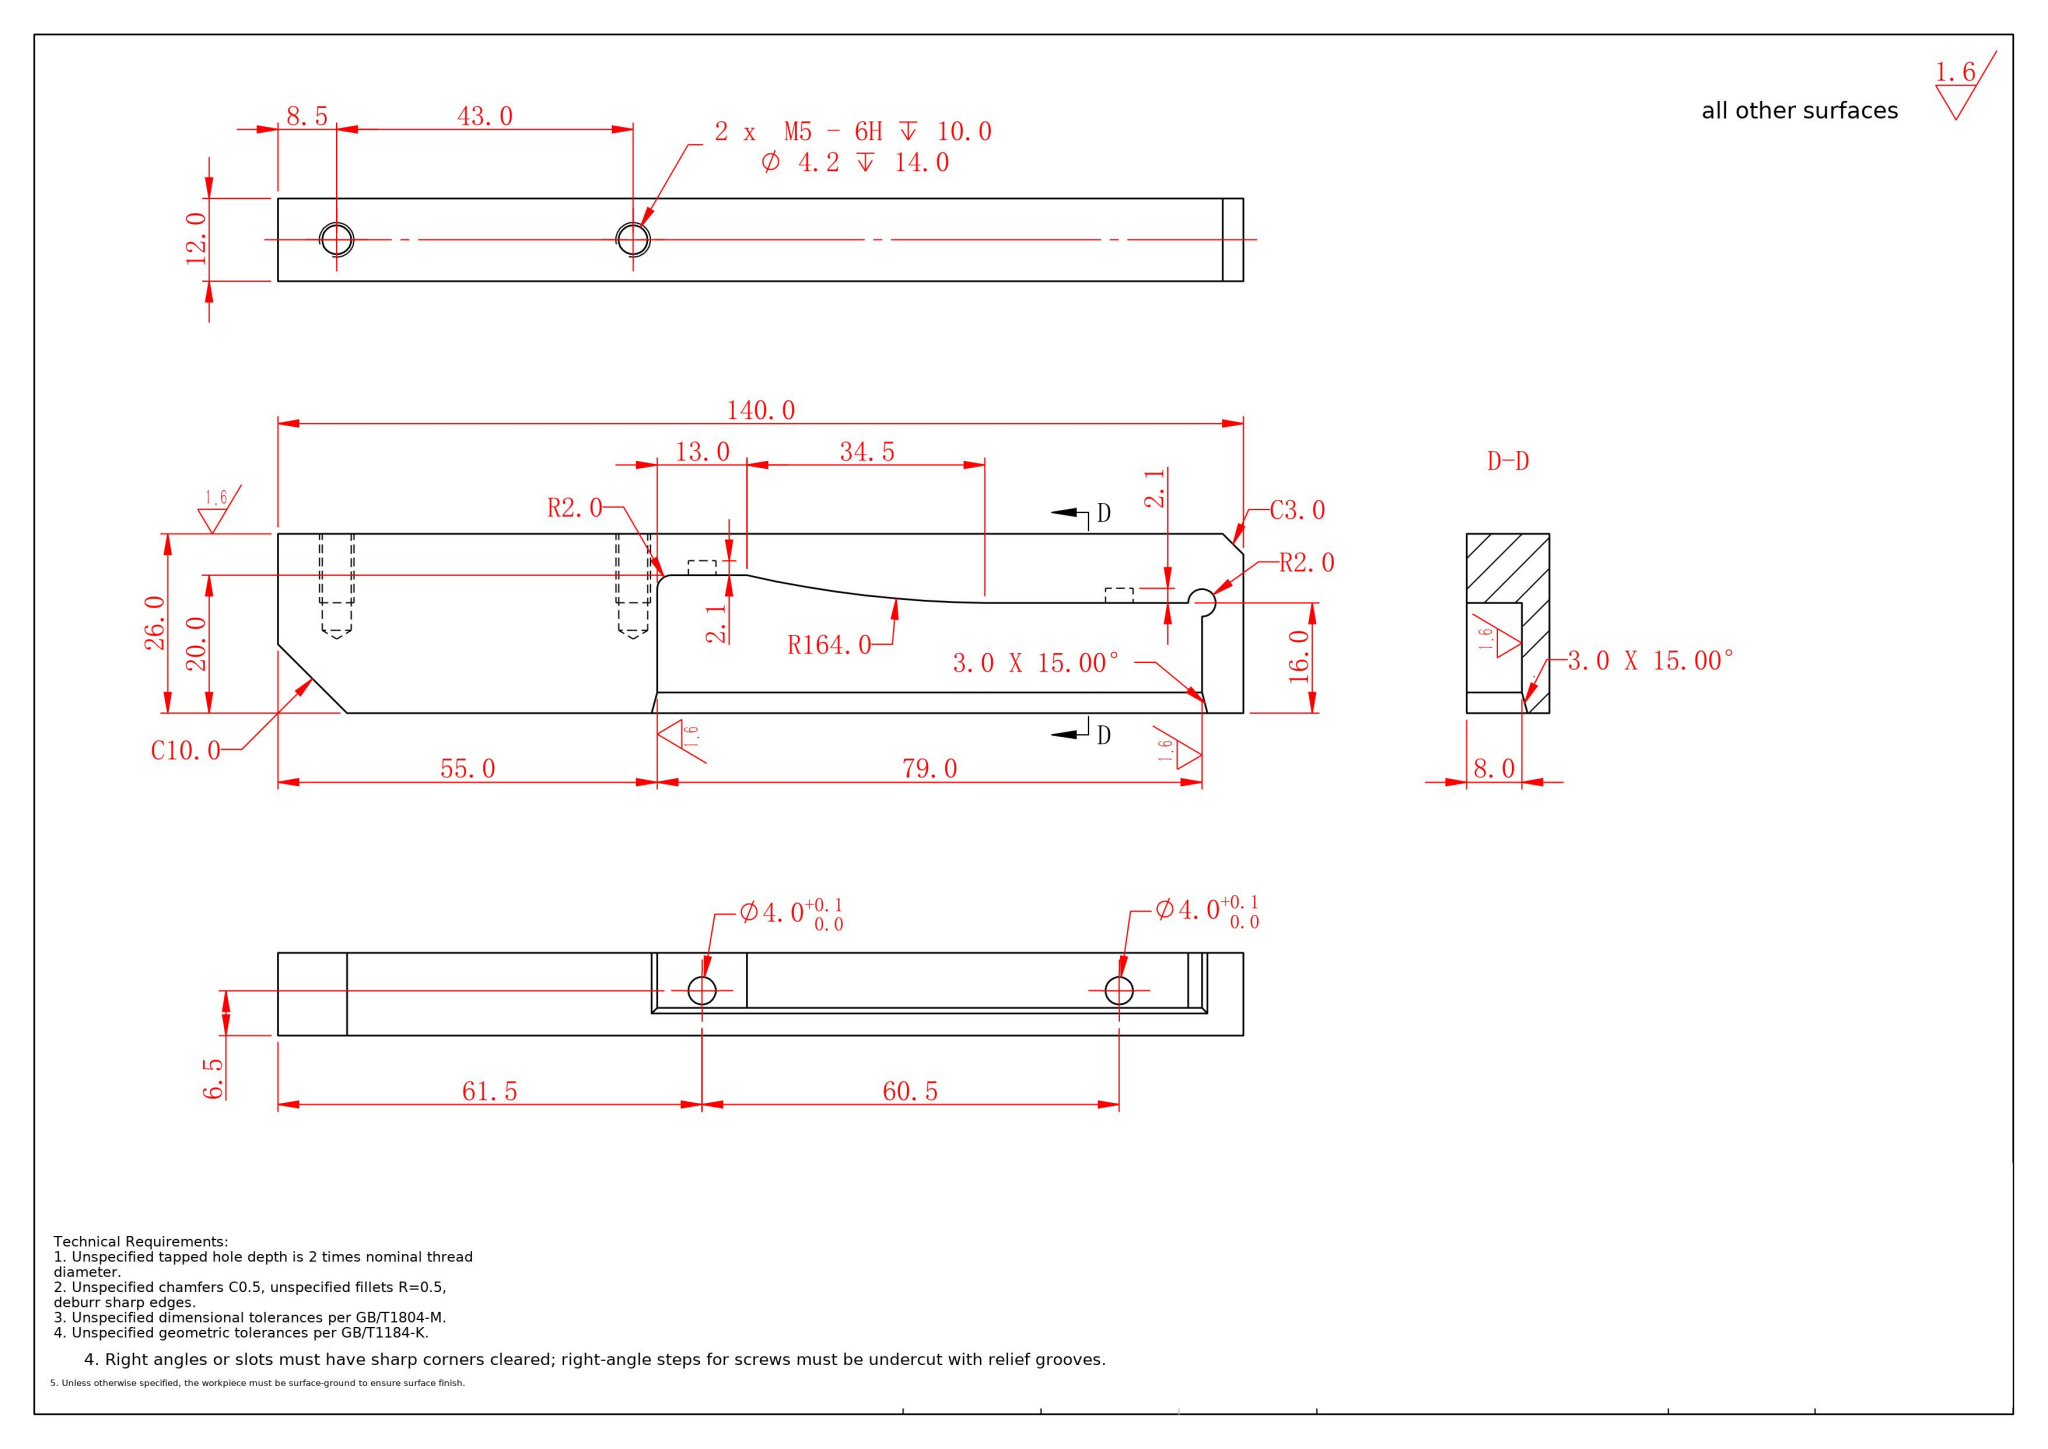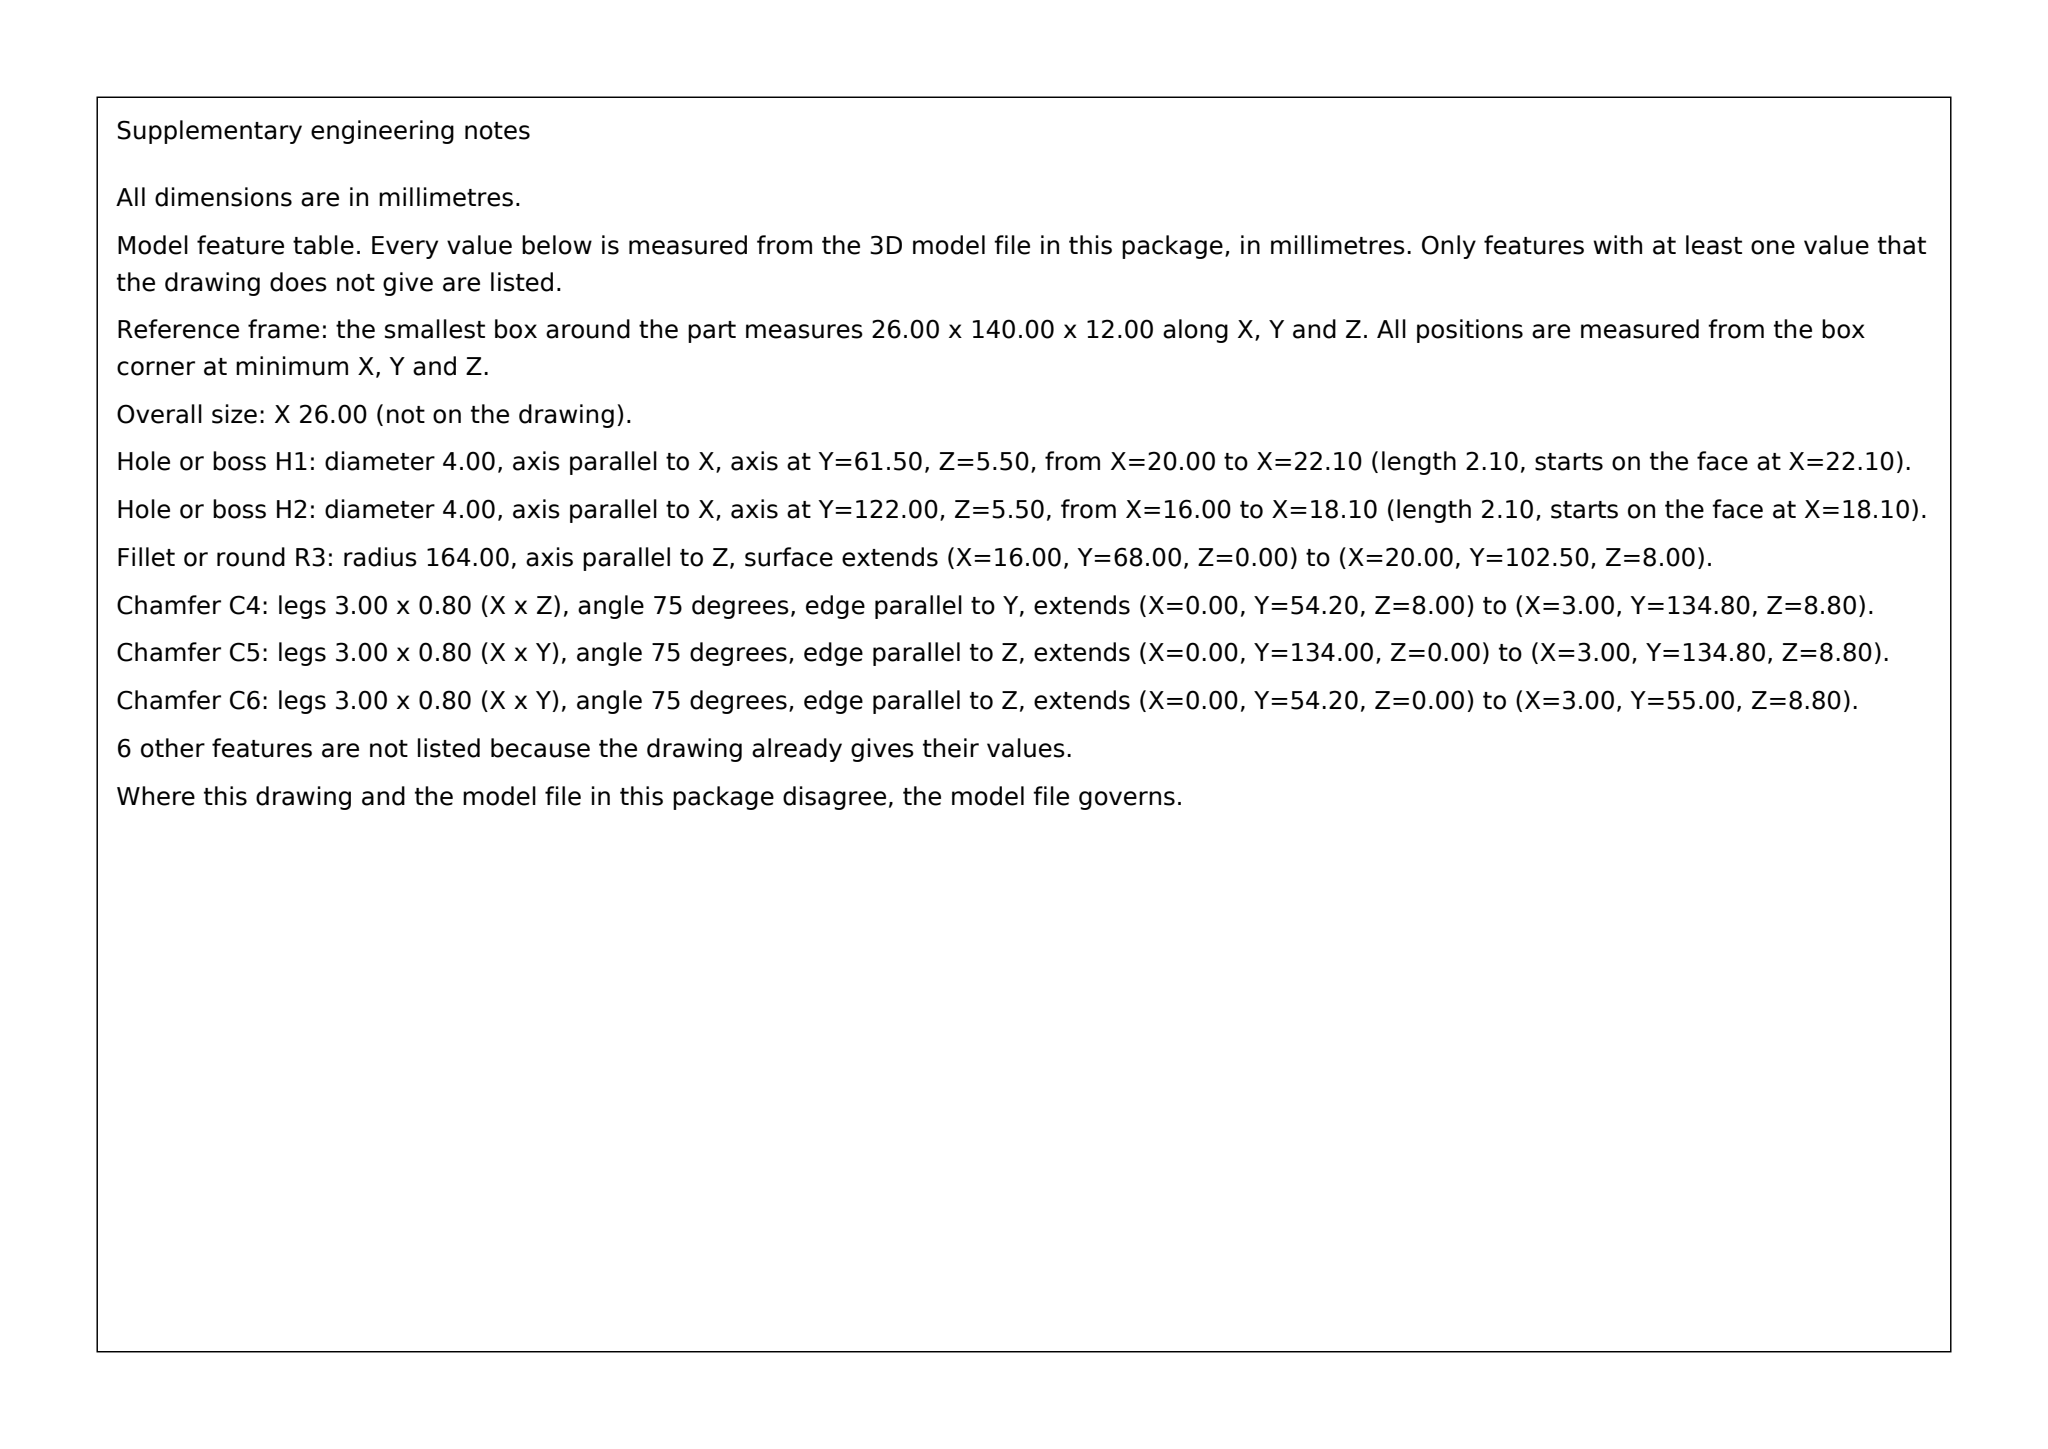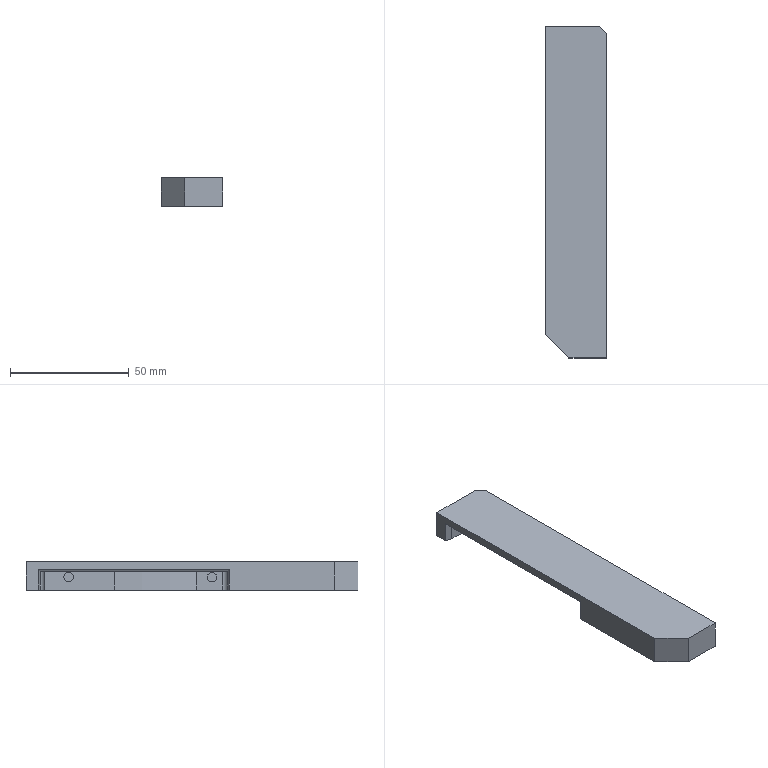Part | SolidWorks | mm | 1 solid | 33 faces | box 26 x 140 x 12 mm | volume 31480 mm3 | plane 18 | cylinder 11 | cone 4 | commonest cylinder face diameters 4 x6 4.2 x4 328 x1
build123d program:
from build123d import *
from OCP.BRepFilletAPI import BRepFilletAPI_MakeChamfer

# Parameters (mm, degrees)
SKETCH1_W             = 26
SKETCH1_H             = 140
BOSS_EXTRUDE1_DEPTH   = 12
CUT_EXTRUDE2_DEPTH    = 8
SKETCH4_R             = 2
CUT_EXTRUDE3_DEPTH    = 2.1
SKETCH5_R             = 2
CUT_EXTRUDE4_DEPTH    = 2.1
FILLET1_R             = 2
SKETCH6_R             = 2
CUT_EXTRUDE5_DEPTH    = 8
CHAMFER1_SIZE         = 3
CHAMFER1_SIZE2        = 0.8038
M5_TAPPED_HOLE1_D     = 4.2
M5_TAPPED_HOLE1_DEPTH = 14
M5_TAPPED_HOLE1_TIP   = 1.262
CHAMFER2_SIZE         = 10
CHAMFER3_SIZE         = 3


with BuildPart() as part:
    # Sketch1 → Boss-Extrude1 (new body)
    with BuildSketch(Plane.XY):
        with Locations((13, 70)):
            Rectangle(SKETCH1_W, SKETCH1_H)
    extrude(amount=BOSS_EXTRUDE1_DEPTH)

    # Sketch3 → Cut-Extrude2 (cut)
    with BuildSketch(Plane(origin=(0, 0, 0), x_dir=(-1, 0, 0), z_dir=(0, 0, -1))):
        with BuildLine():
            Line((-16, 134), (-16, 102.5))
            ThreePointArc((-16, 102.5), (-17.084, 85.144), (-20, 68))
            Line((-20, 68), (-20, 55))
            Line((-20, 55), (0, 55))
            Line((0, 55), (0, 134))
            Line((0, 134), (-16, 134))
        make_face()
    extrude(amount=-CUT_EXTRUDE2_DEPTH, mode=Mode.SUBTRACT)

    # Sketch4 → Cut-Extrude3 (cut)
    with BuildSketch(Plane.ZY.offset(-20)):
        with Locations(Location((5.5, 61.5, 0), (0, 0, 270))):
            Circle(SKETCH4_R)
    extrude(amount=-CUT_EXTRUDE3_DEPTH, mode=Mode.SUBTRACT)

    # Sketch5 → Cut-Extrude4 (cut)
    with BuildSketch(Plane.ZY.offset(-16)):
        with Locations((5.5, 122)):
            Circle(SKETCH5_R)
    extrude(amount=-CUT_EXTRUDE4_DEPTH, mode=Mode.SUBTRACT)

    # Fillet1
    fillet1_edges = [part.edges().sort_by_distance(p)[0] for p in [
        (20, 55, 4),
    ]]
    fillet(fillet1_edges, radius=FILLET1_R)

    # Sketch6 → Cut-Extrude5 (cut)
    with BuildSketch(Plane(origin=(0, 0, 0), x_dir=(-1, 0, 0), z_dir=(0, 0, -1))):
        with Locations((-16, 134)):
            Circle(SKETCH6_R)
    extrude(amount=-CUT_EXTRUDE5_DEPTH, mode=Mode.SUBTRACT)

    # Chamfer1: one chamfer whose edges measure the first distance from different faces: ONE call of the kernel's chamfer builder (chamfer() names one face for all edges)
    chamfer1_edges_1 = [part.edges().sort_by_distance(p)[0] for p in [
        (0, 94.5, 8),
    ]]
    chamfer1_side_1 = [part.faces().sort_by_distance(p)[0] for p in [
        (8.748, 92.938, 8),
    ]]
    chamfer1_edges_2 = [part.edges().sort_by_distance(p)[0] for p in [
        (0, 134, 4),
    ]]
    chamfer1_side_2 = [part.faces().sort_by_distance(p)[0] for p in [
        (7, 134, 4),
    ]]
    chamfer1_edges_3 = [part.edges().sort_by_distance(p)[0] for p in [
        (0, 55, 4),
    ]]
    chamfer1_side_3 = [part.faces().sort_by_distance(p)[0] for p in [
        (9, 55, 4),
    ]]
    chamfer1 = BRepFilletAPI_MakeChamfer(part.part.solid().wrapped)
    for e in chamfer1_edges_1:
        chamfer1.Add(CHAMFER1_SIZE, CHAMFER1_SIZE2, e.wrapped, chamfer1_side_1[0].wrapped)  # the first distance lies on this face
    for e in chamfer1_edges_2:
        chamfer1.Add(CHAMFER1_SIZE, CHAMFER1_SIZE2, e.wrapped, chamfer1_side_2[0].wrapped)  # the first distance lies on this face
    for e in chamfer1_edges_3:
        chamfer1.Add(CHAMFER1_SIZE, CHAMFER1_SIZE2, e.wrapped, chamfer1_side_3[0].wrapped)  # the first distance lies on this face
    add(Compound.cast(chamfer1.Shape()), mode=Mode.REPLACE)

    # M5 Tapped Hole1
    with Locations(Plane(origin=(26, 0, 0), x_dir=(0, 0, -1), z_dir=(1, 0, 0))):
        with Locations((-6, 51.5), (-6, 8.5)):
            Hole(M5_TAPPED_HOLE1_D / 2, depth=M5_TAPPED_HOLE1_DEPTH)
            with Locations((0, 0, -(M5_TAPPED_HOLE1_DEPTH + M5_TAPPED_HOLE1_TIP / 2))):  # 118° drill point
                Cone(0, M5_TAPPED_HOLE1_D / 2, M5_TAPPED_HOLE1_TIP, mode=Mode.SUBTRACT)

    # Chamfer2
    chamfer2_edges = [part.edges().sort_by_distance(p)[0] for p in [
        (0, 0, 6),
    ]]
    chamfer(chamfer2_edges, length=CHAMFER2_SIZE)

    # Chamfer3
    chamfer3_edges = [part.edges().sort_by_distance(p)[0] for p in [
        (26, 140, 6),
    ]]
    chamfer(chamfer3_edges, length=CHAMFER3_SIZE)


solid = part.part